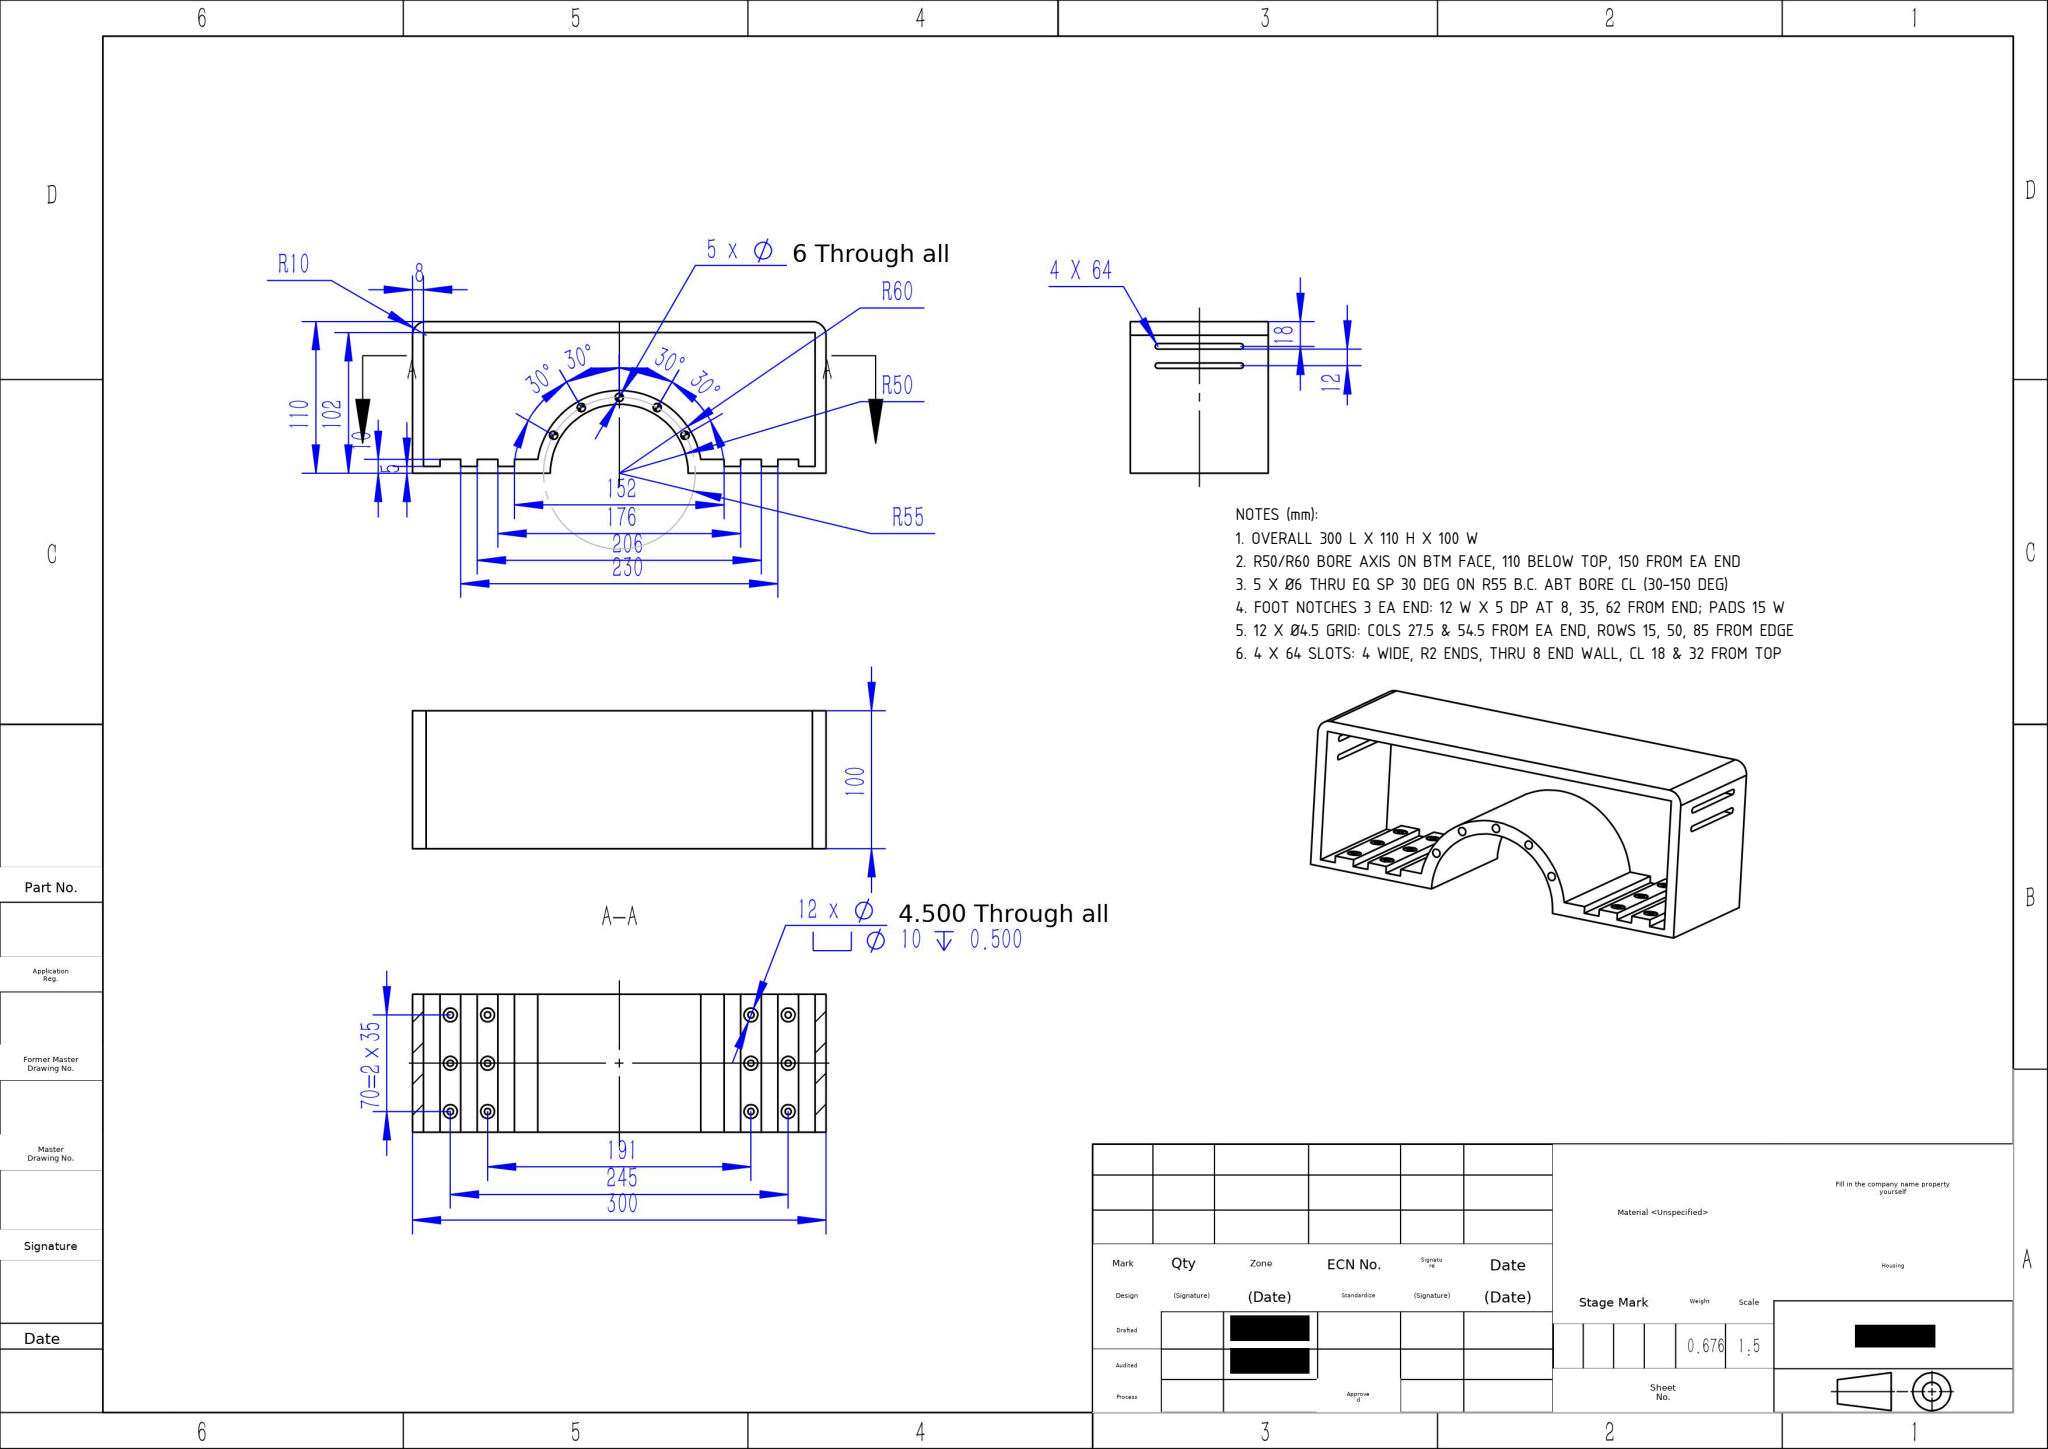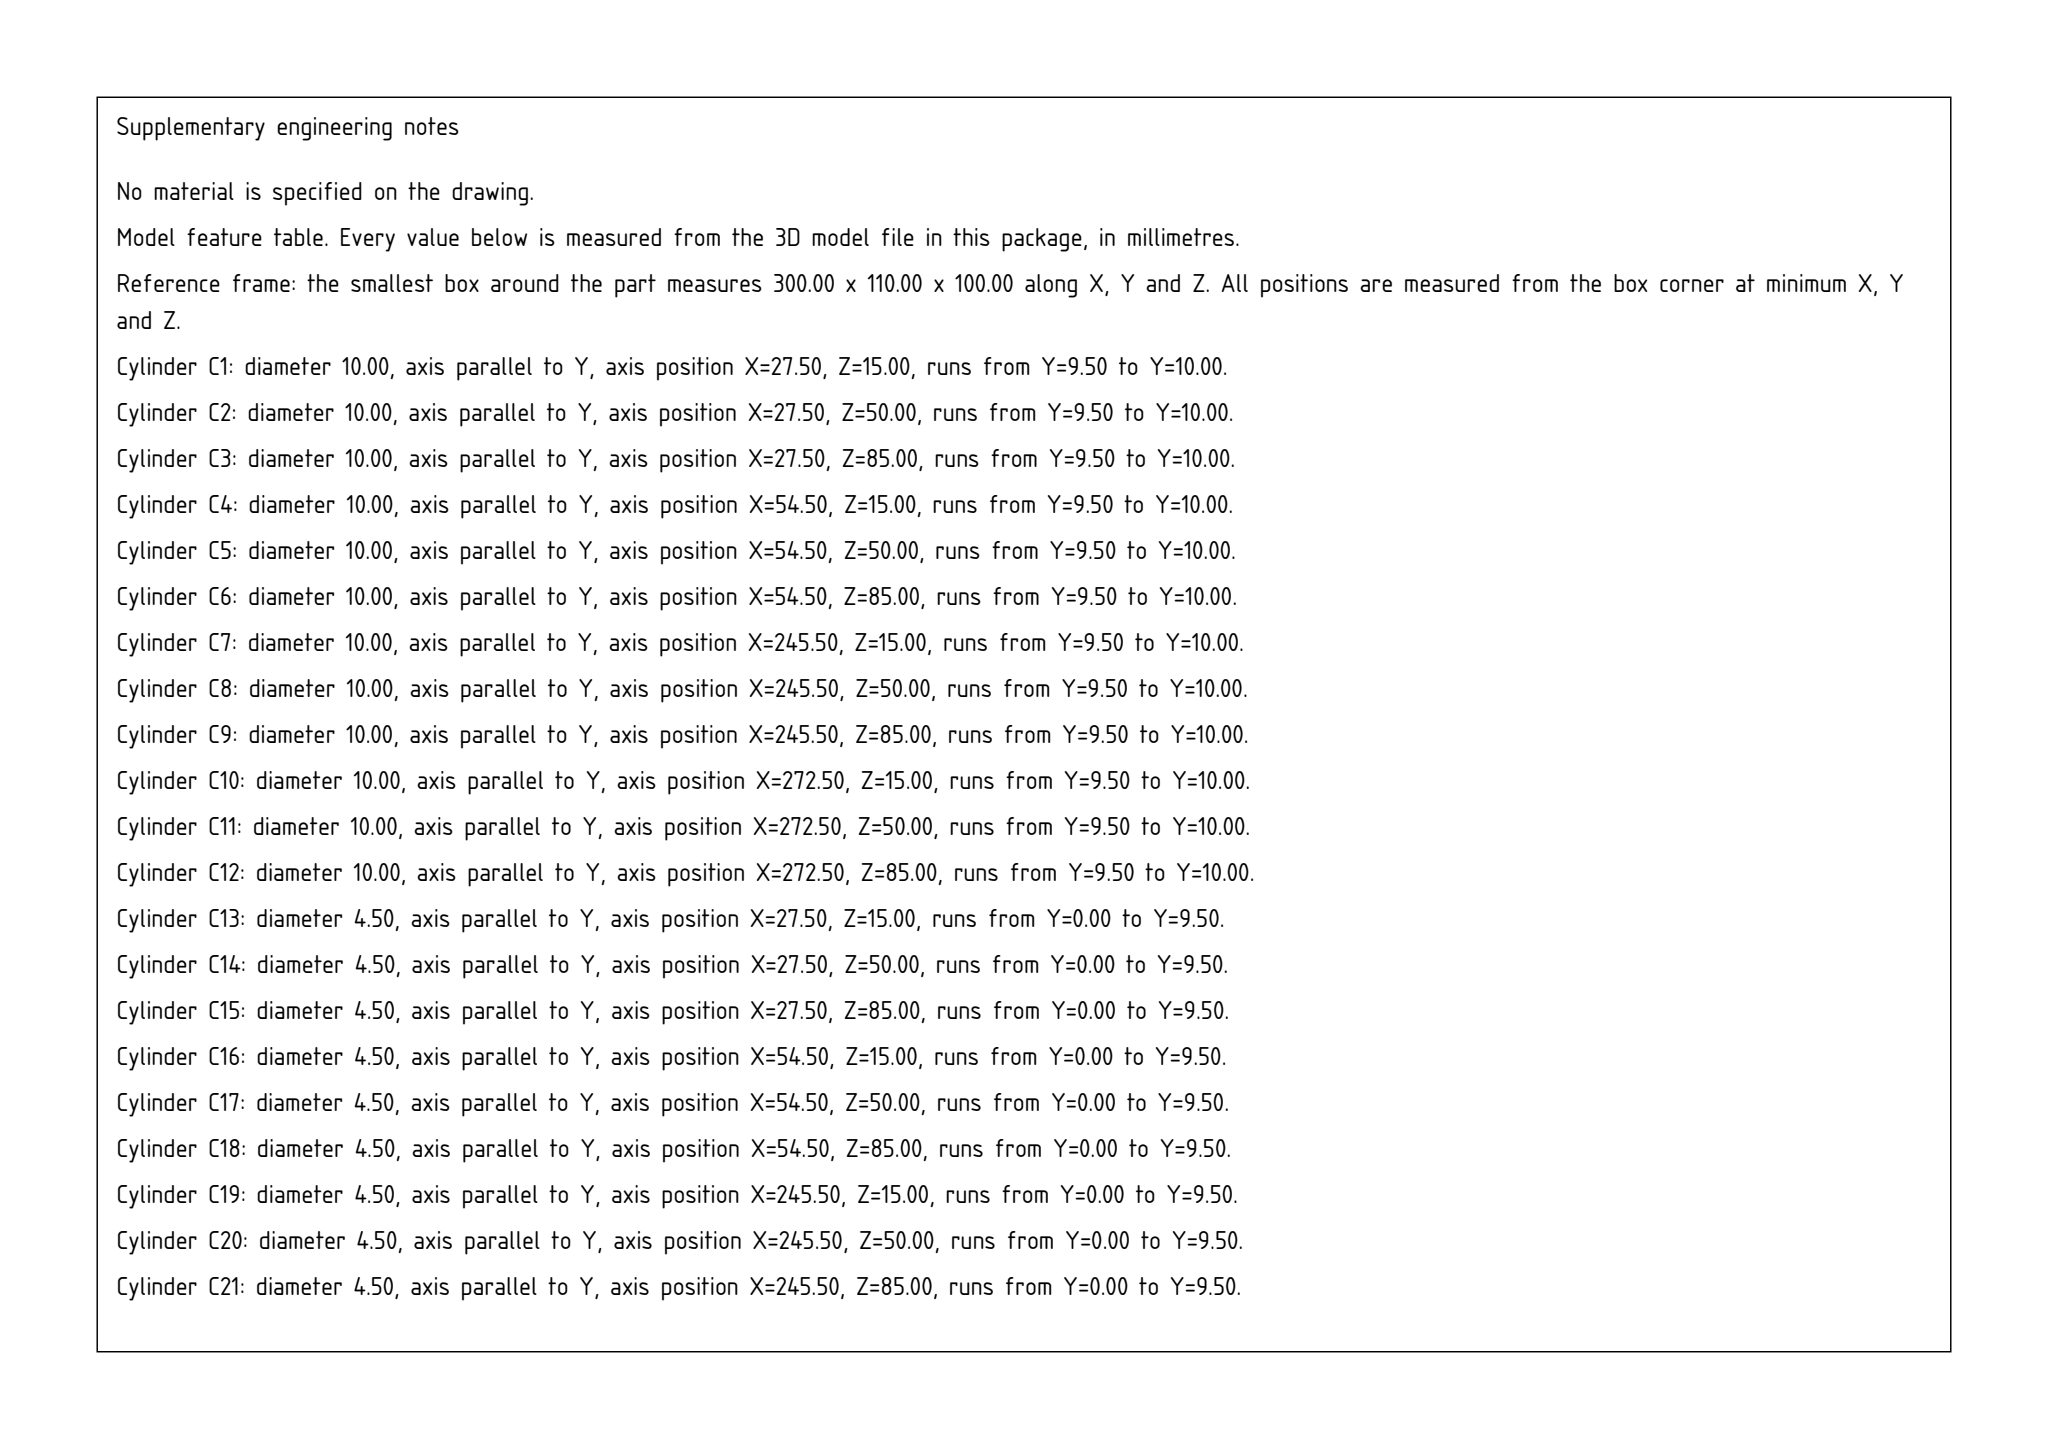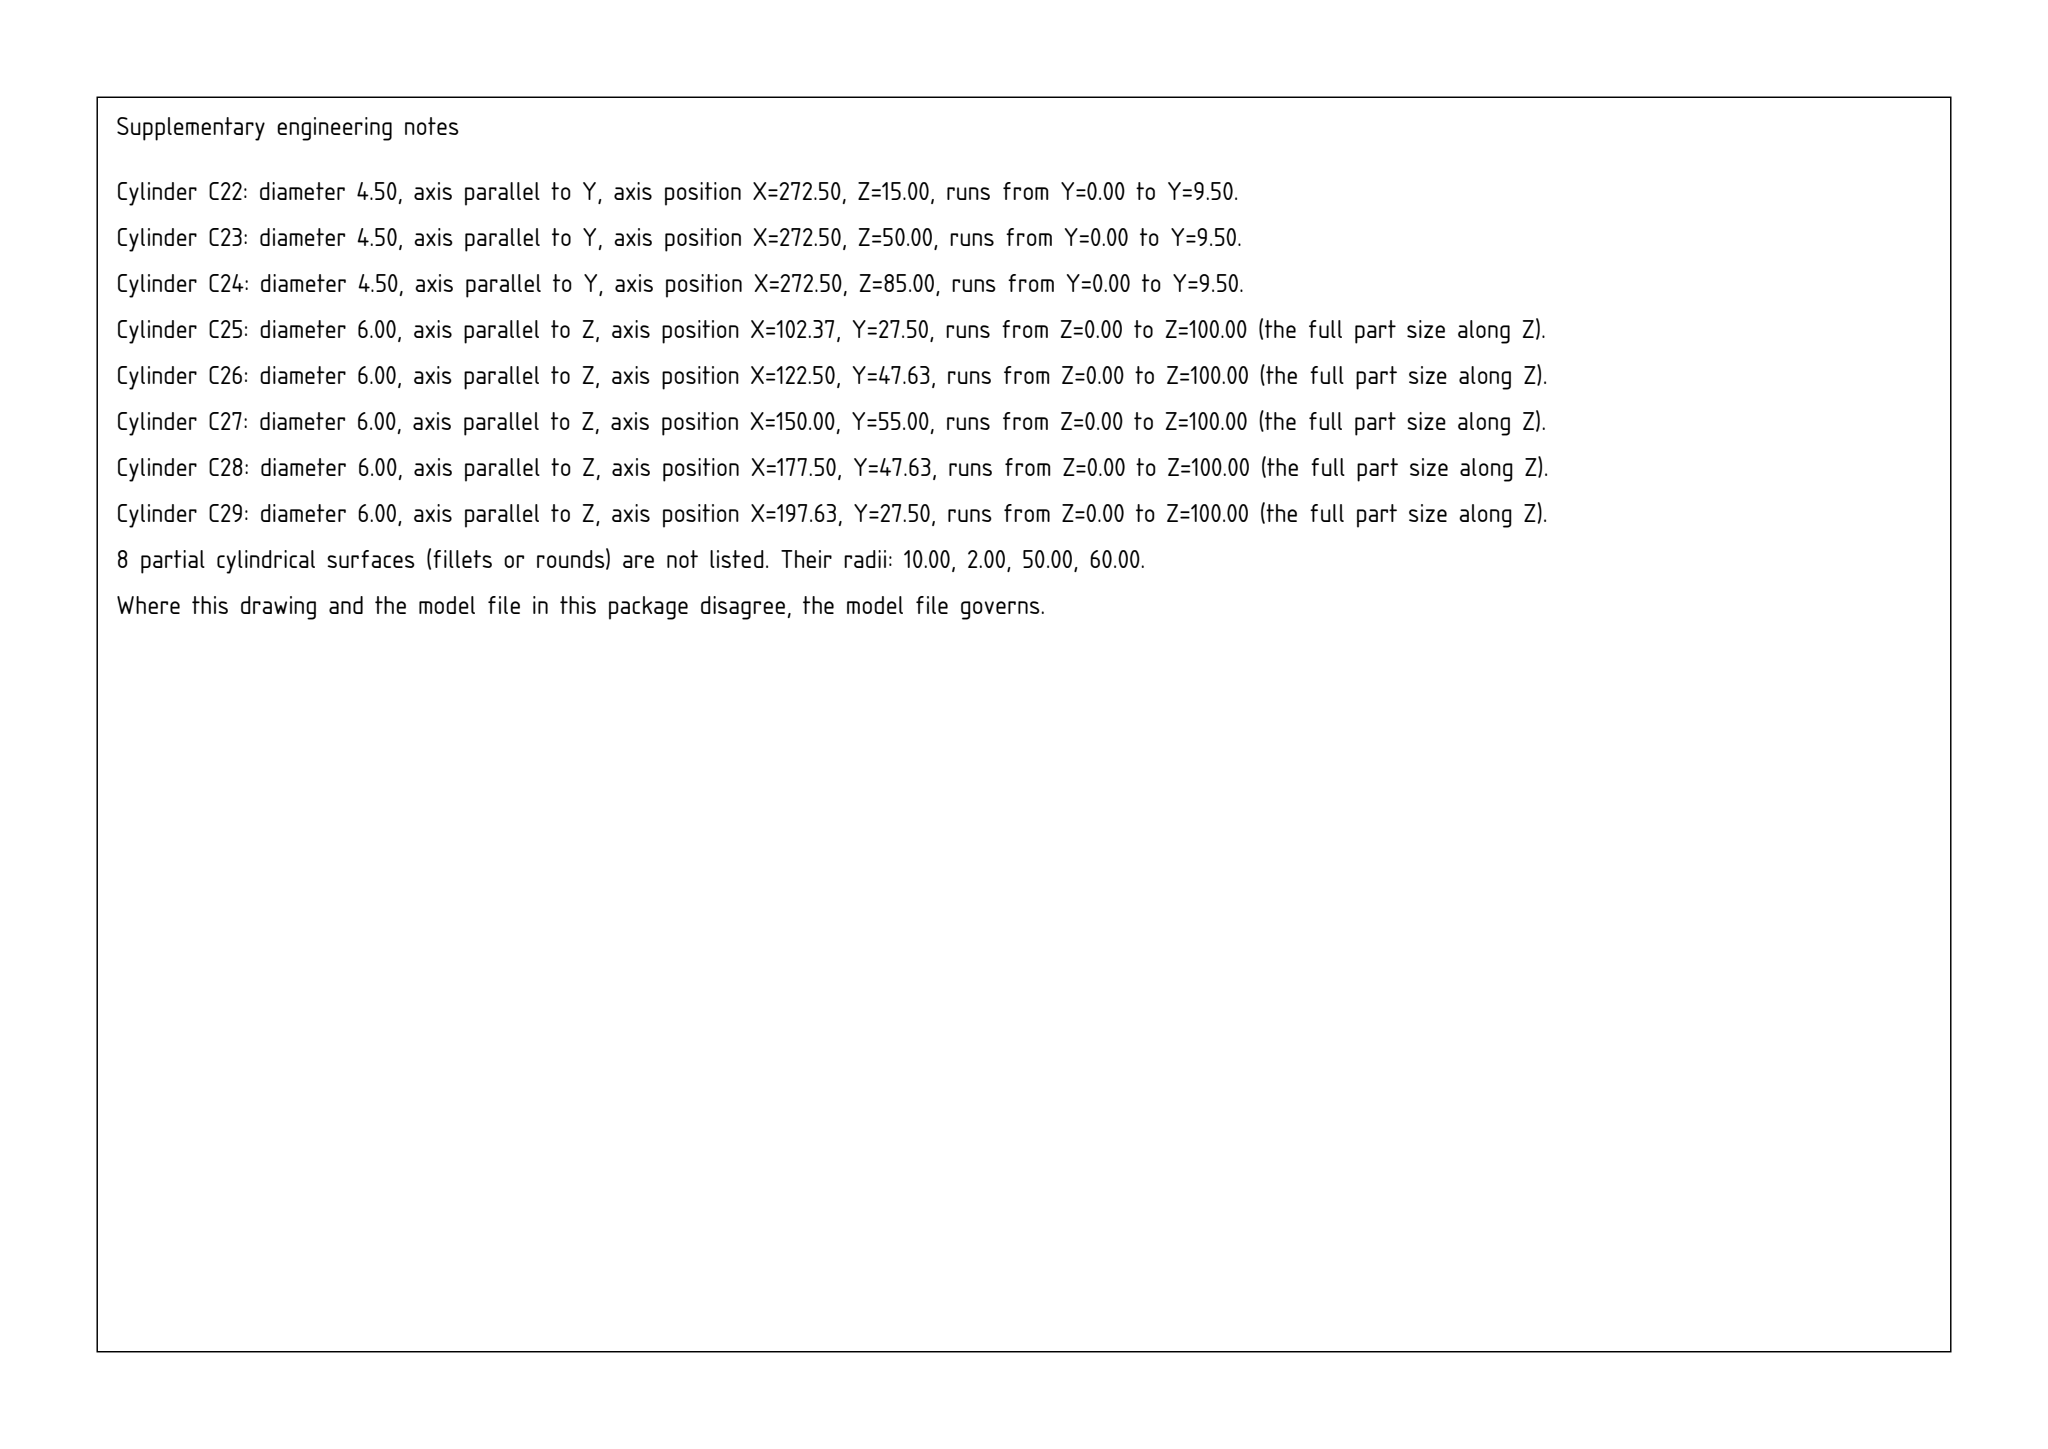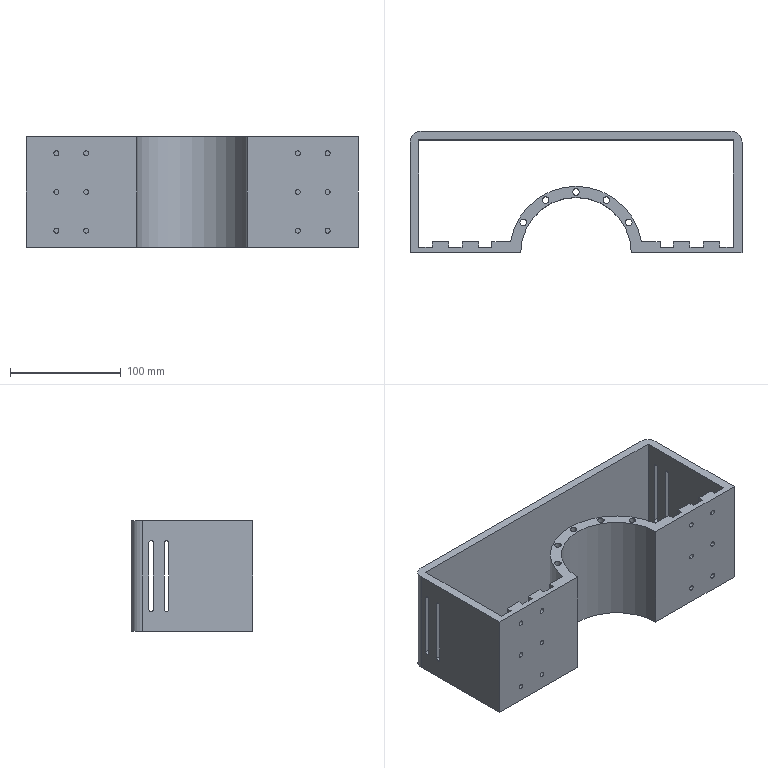Part | SolidWorks | mm | 1 solid | 126 faces | box 300 x 110 x 100 mm | volume 675750 mm3 | cylinder 74 | plane 52 | commonest cylinder face diameters 10 x24 4.5 x24 4 x12 6 x10 20 x2 120 x1 100 x1
Drawing notes:
OVERALL 300 L X 110 H X 100 W | from the solid: bbox_xyz 300.0 x 110.0 x 100.0
R50/R60 BORE AXIS ON BTM FACE, 110 BELOW TOP, 150 FROM EA END | from the solid: Ø100 & Ø120 z-axis cyls at (x=150.0, y=0.0), L=100; bbox height 110
5 X Ø6 THRU EQ SP 30 DEG ON R55 B.C. ABT BORE CL (30-150 DEG) | from the solid: Ø6 z-holes at (102.37,27.5),(122.5,47.63),(150,55),(177.5,47.63),(197.63,27.5), all R55 from (150,0)
FOOT NOTCHES 3 EA END: 12 W X 5 DP AT 8, 35, 62 FROM END; PADS 15 W | from the solid: x-planes 8,20,35,47,62,74 and mirror 226,238,253,265,280,292; notch floors y=5, foot y=0-10
12 X Ø4.5 GRID: COLS 27.5 & 54.5 FROM EA END, ROWS 15, 50, 85 FROM EDGE | from the solid: Ø4.5 y-holes at x=27.5,54.5,245.5,272.5 and z=15,50,85, L=9.5 with Ø10 x 0.5 CBORE
4 X 64 SLOTS: 4 WIDE, R2 ENDS, THRU 8 END WALL, CL 18 & 32 FROM TOP | from the solid: Ø4 x-axis cyls L=8 at (y78,z20),(y78,z80),(y92,z20),(y92,z80); wall planes x=0/8, top y=110
build123d program:
from build123d import *

# Parameters (mm, degrees)
EXTRUDE_THIN1_DEPTH                       = 50
SKETCH2_W                                 = 12
SKETCH2_H                                 = 100
CUT_EXTRUDE1_DEPTH                        = 5
F_6_0MM_DOWEL_PIN_HOLE1_D                 = 6
BOSS_EXTRUDE1_DEPTH                       = 100
M4_HEX_HEAD_BOLT_COUNTERBORE1_D           = 4.5
M4_HEX_HEAD_BOLT_COUNTERBORE1_DEPTH       = 10
M4_HEX_HEAD_BOLT_COUNTERBORE1_CBORE_D     = 10
M4_HEX_HEAD_BOLT_COUNTERBORE1_CBORE_DEPTH = 0.5
FILLET1_R                                 = 10
CUT_EXTRUDE2_DEPTH                        = 324.419


with BuildPart() as part:
    # Sketch1 → Extrude-Thin1 (new, symmetric)
    with BuildSketch(Plane.XY):
        with BuildLine():
            Line((150, 0), (50, 0))
            ThreePointArc((50, 0), (0, 50), (-50, 0))
            Line((-50, 0), (-150, 0))
            Line((-150, 0), (-150, 10))
            Line((-150, 10), (-59.161, 10))
            ThreePointArc((-59.161, 10), (0, 60), (59.161, 10))
            Line((59.161, 10), (150, 10))
            Line((150, 10), (150, 0))
        make_face()
    extrude(amount=EXTRUDE_THIN1_DEPTH, both=True)

    # Sketch2 → Cut-Extrude1 (cut)
    with BuildSketch(Plane(origin=(0, 10, 0), x_dir=(1, 0, 0), z_dir=(0, 1, 0))):
        with Locations((-136, 0)):
            Rectangle(SKETCH2_W, SKETCH2_H)
        with Locations((-109, 0)):
            Rectangle(SKETCH2_W, SKETCH2_H)
        with Locations((-82, 0)):
            Rectangle(SKETCH2_W, SKETCH2_H)
        with Locations((82, 0)):
            Rectangle(SKETCH2_W, SKETCH2_H)
        with Locations((109, 0)):
            Rectangle(SKETCH2_W, SKETCH2_H)
        with Locations((136, 0)):
            Rectangle(SKETCH2_W, SKETCH2_H)
    extrude(amount=-CUT_EXTRUDE1_DEPTH, mode=Mode.SUBTRACT)

    # 6.0mm Dowel Pin Hole1 (through all)
    with Locations(Plane.XY.offset(50)):
        with Locations((27.5, 47.631), (0, 55), (-27.5, 47.631), (-47.631, 27.5), (47.631, 27.5)):
            Hole(F_6_0MM_DOWEL_PIN_HOLE1_D / 2)

    # Sketch6 → Boss-Extrude1 (add)
    with BuildSketch(Plane.XY.offset(50)):
        Polygon((-150, 10), (-150, 110), (150, 110), (150, 10), (142, 10), (142, 102), (-142, 102), (-142, 10), align=None)
    extrude(amount=-BOSS_EXTRUDE1_DEPTH)

    # M4 Hex Head Bolt Counterbore1
    with Locations(Plane(origin=(0, 10, 0), x_dir=(1, 0, 0), z_dir=(0, 1, 0))):
        with Locations((-122.5, 35), (-122.5, 0), (-122.5, -35), (-95.5, 35), (-95.5, 0), (-95.5, -35), (95.5, -35), (95.5, 0), (95.5, 35), (122.5, -35), (122.5, 0), (122.5, 35)):
            CounterBoreHole(M4_HEX_HEAD_BOLT_COUNTERBORE1_D / 2, M4_HEX_HEAD_BOLT_COUNTERBORE1_CBORE_D / 2, M4_HEX_HEAD_BOLT_COUNTERBORE1_CBORE_DEPTH, depth=M4_HEX_HEAD_BOLT_COUNTERBORE1_DEPTH)

    # Fillet1
    fillet1_edges = [part.edges().sort_by_distance(p)[0] for p in [
        (-150, 110, 0),
        (150, 110, 0),
    ]]
    fillet(fillet1_edges, radius=FILLET1_R)

    # Sketch11 → Cut-Extrude2 (cut, through all)
    with BuildSketch(Plane.ZY.offset(150)):
        with BuildLine():
            Line((-30, 94), (30, 94))
            ThreePointArc((30, 94), (32, 92), (30, 90))
            Line((30, 90), (-30, 90))
            ThreePointArc((-30, 90), (-32, 92), (-30, 94))
        make_face()
        with BuildLine():
            Line((-30, 80), (30, 80))
            ThreePointArc((30, 80), (32, 78), (30, 76))
            Line((30, 76), (-30, 76))
            ThreePointArc((-30, 76), (-32, 78), (-30, 80))
        make_face()
    extrude(amount=-CUT_EXTRUDE2_DEPTH, mode=Mode.SUBTRACT)


solid = part.part